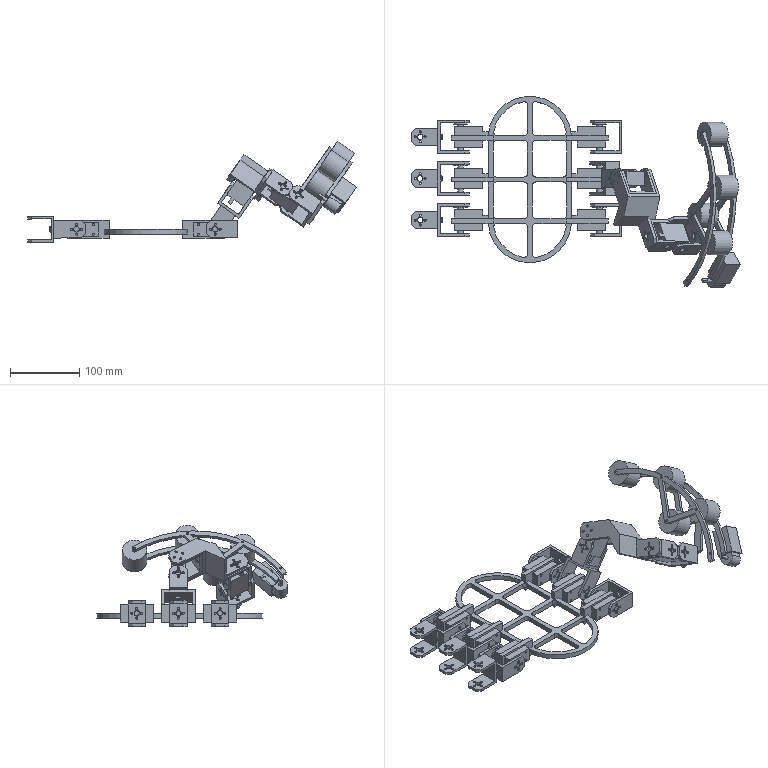Assembly | NX | mm | 33 component files | 41 solids | 871 faces | box 474.04 x 275.69 x 145.87 mm | volume 665786 mm3 | plane 498 | cylinder 350 | other 17 | cone 6 | commonest cylinder face diameters 3 x227 8 x59 10 x28 20 x11 300 x6 35 x4 106 x4 120 x2
Bill of materials:
unnamed part 1 | 3 |  | Solid right circular cylinder with a chamfer on the edge at each end; flat circular end faces; length somewhat greater than diameter.
unnamed part 2 | 1 |  | Bracket made of thin plates: a rectangular box-like central section with two parallel arms with chamfered ends extending one way, and a single arm extending the opposite way. The arm ends have small hole patterns.
unnamed part 3 | 1 |  | Thin, flat, curved arc-shaped strip with a V-shaped brace on its concave side that connects two points of the arc. Small holes at the arc ends, the brace junctions and the V apex.
unnamed part 4 | 1 |  | Block-like body with one rounded (semicircular) end. A short cylindrical boss with a flat end sits on one face near the square end, and a slender shaft projects from the rounded end. The shaft has a stepped or flat-cut section near its tip, and the body has two through-holes.
unnamed part 5 | 4 |  | Solid cylinder, diameter roughly equal to or larger than its length, with one small hole on the axis of a flat end face.
unnamed part 6 | 1 |  | Flat lattice/grid frame: an obround (stadium-shaped) outer ring with an internal cross-grid of ribs. Three parallel straight bars extend outward on both sides, each ending in a raised rectangular open frame (rectangular loop).
unnamed part 7 | 8 |  | U-shaped (channel) bracket of constant-thickness plate. The two side flanges have chamfered free corners, and each of the three faces has a hole pattern of one large center hole with four smaller holes around it.
unnamed part 8 | 1 |  | Arc-shaped strip with a V-shaped brace (similar to a curved truss segment), combined with a rectangular block near one end and an angled bent-plate (V/L-shaped) extension.
unnamed part 9 | 5 |  | U-shaped (channel) bracket of uniform plate. Both flanges and the web each have a central large hole with four smaller holes in a cross pattern. One flange view shows a chamfered-corner outline.
unnamed part 10 | 8 |  | Rectangular block body with stepped/offset sections and a projecting tab, a circular flange disc with four holes on one side face, and a short cylindrical shaft/boss projecting from an end.
Mates:
1. fix | bottom_cover 1 component
2. touch align | servo 8 face | bottom_cover 1 face
3. touch align | servo 8 face | bottom_cover 1 face
4. touch align | servo 5 face | bottom_cover 1 face
5. touch align | servo 5 face | bottom_cover 1 face
6. touch align | servo 5 face | bottom_cover 1 face
7. touch align | servo 6 face | bottom_cover 1 face
8. touch align | servo 6 face | bottom_cover 1 face
9. touch align | servo 6 face | bottom_cover 1 face
10. touch align | servo 7 face | bottom_cover 1 face
11. touch align | servo 7 face | bottom_cover 1 face
12. touch align | servo 7 face | bottom_cover 1 face
13. touch align | servo 4 face | bottom_cover 1 face
14. touch align | servo 4 face | bottom_cover 1 face
15. touch align | servo 4 face | bottom_cover 1 face
16. touch align | servo 3 face | bottom_cover 1 face
17. touch align | servo 3 face | bottom_cover 1 face
18. touch align | servo 3 face | bottom_cover 1 face
19. concentric | U_shape 8 edge | servo 8 edge
20. touch align | bottom_cover 1 face | servo 8 face
21. concentric | U_shape 6 edge | servo 4 edge
22. concentric | U_shape 5 edge | servo 3 edge
23. concentric | U_shape 4 edge | servo 5 edge
24. concentric | U_shape 3 edge | servo 6 edge
25. concentric | U_shape 7 edge | servo 7 edge
26. concentric | lower_leg 1 edge | sprocket 4 edge
27. touch align | sprocket 2 face | lower_leg 1 face
28. concentric | lower_leg_2 1 edge | sprocket 2 edge
29. touch align | lower_leg_2 1 face | sprocket 3 face
30. concentric | U_shape_2 5 edge | U_shape 6 edge
31. touch align | servo 2 face | U_shape_2 5 face
32. touch align | U_shape_2 5 face | U_shape 6 face
33. touch align | U_shape 2 face | servo 2 face
34. touch align | U_shape 2 face | servo 2 face
35. touch align | U_shape_3 1 face | U_shape 2 face
36. touch align | U_shape_3 1 face | U_shape 2 face
37. touch align | U_shape 2 face | U_shape_3 1 face
38. distance | U_shape_2 5 face | servo 2 face
39. touch align | U_shape_2 5 face | servo 2 face
40. touch align | servo 2 face | U_shape_2 5 face
41. concentric | servo 1 edge | U_shape_2 4 edge
42. touch align | U_shape_2 4 face | servo 1 face
43. concentric | U_shape 1 edge | servo 1 edge
44. concentric | U_shape_2 4 edge | U_shape_3 1 edge
45. touch align | U_shape_2 4 face | U_shape_3 1 face
46. touch align | lower_leg 1 face | motor 1 face
47. concentric | sprocket 1 edge | lower_leg_2 1 edge
48. touch align | motor 1 face | lower_leg 1 face
49. touch align | motor 1 face | lower_leg 1 face
50. concentric | sprocket 1 edge | lower_leg 1 edge
51. concentric | sprocket 3 edge | lower_leg 1 edge
52. touch align | lower_leg 1 face | U_shape 1 face
53. concentric | U_shape_2 3 edge | U_shape 3 edge
54. touch align | U_shape 3 face | U_shape_2 3 face
55. concentric | U_shape_2 2 edge | U_shape 4 edge
56. concentric | U_shape 7 edge | U_shape_2 1 edge
57. touch align | U_shape_2 2 face | U_shape 4 face
58. touch align | U_shape_2 3 face | U_shape 3 face
59. touch align | locating_pin 3 face | U_shape_2 2 face
60. distance | locating_pin 3 face | U_shape_2 2 face
61. fix | assembly component
62. bond | locating_pin 3 component | assembly component
63. bond | locating_pin 2 component | assembly component
64. linear | assembly datumaxis | assembly cartesiancoordinatesystem | assembly cartesiancoordinatesystem | assembly cartesiancoordinatesystem
65. bond | locating_pin 1 component | assembly component